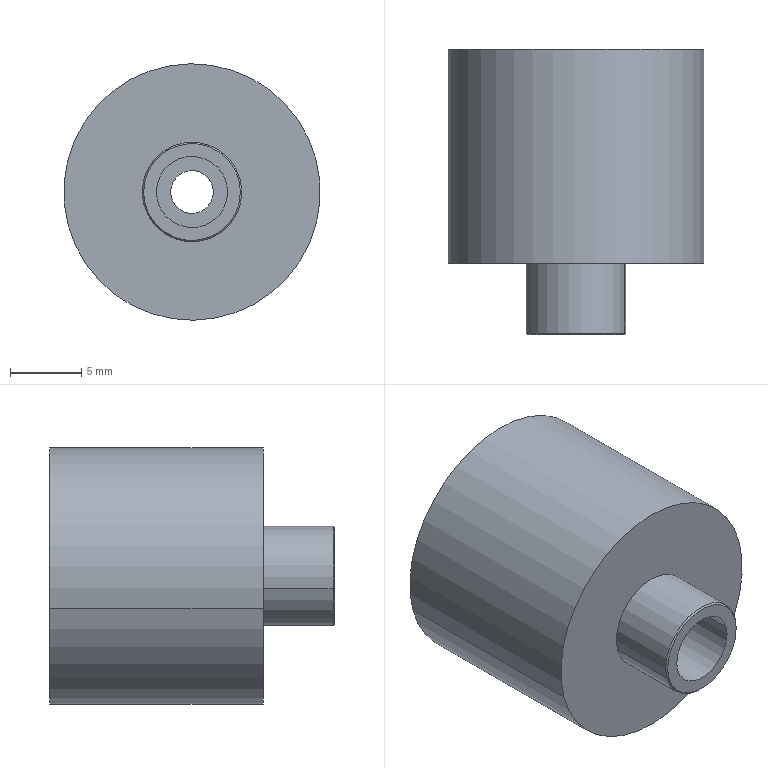Component | SolidWorks | WireFeedingConnector-1 | 1 solid | 19 faces | box 18 x 20 x 18 mm | volume 3059 mm3 | cylinder 10 | plane 5 | cone 4 | commonest cylinder face diameters 5 x2 10 x2 18 x2 7 x2 3 x2
build123d program:
from build123d import *

# Parameters (mm, degrees)
CHAMFER1_SIZE      = 0.1
CHAMFER2_SIZE      = 0.1
SKETCH1_R          = 2.5
CUT_EXTRUDE1_DEPTH = 7.5


with BuildPart() as part:
    # Sketch1_2 → Revolve1 (revolve)
    with BuildSketch(Plane.XY, mode=Mode.PRIVATE) as revolve1_sk:
        Polygon((-1.5, -5), (-3.5, -5), (-3.5, 0), (-9, 0), (-9, 15), (-5, 15), (-5, 5), (-1.5, 5), align=None)
    revolve(revolve1_sk.sketch.rotate(Axis((0, 18.5, 0), (0, -1, 0)), 270), axis=Axis((0, 18.5, 0), (0, -1, 0)))

    # Chamfer1
    chamfer1_edges = [part.edges().sort_by_distance(p)[0] for p in [
        (0, -5, -3.5),
    ]]
    chamfer(chamfer1_edges, length=CHAMFER1_SIZE)

    # Chamfer2
    chamfer2_edges = [part.edges().sort_by_distance(p)[0] for p in [
        (0, 15, -5),
    ]]
    chamfer(chamfer2_edges, length=CHAMFER2_SIZE)

    # Sketch1 → Cut-Extrude1 (cut)
    with BuildSketch(Plane.XZ.offset(5)):
        with Locations(Location((0, 0, 0), (0, 0, 270))):
            Circle(SKETCH1_R)
    extrude(amount=-CUT_EXTRUDE1_DEPTH, mode=Mode.SUBTRACT)


solid = part.part

# Placed as in the assembly
solid = solid.moved(Location((37.32, 90.506, 185), (0, 0, 0)))
STEP:
#1=COLOUR_RGB('',0.7922,0.8196,0.9333);
#2=FILL_AREA_STYLE_COLOUR('',#1);
#3=FILL_AREA_STYLE('',(#2));
#4=SURFACE_STYLE_FILL_AREA(#3);
#5=SURFACE_SIDE_STYLE('',(#4));
#6=SURFACE_STYLE_USAGE(.BOTH.,#5);
#7=PRESENTATION_STYLE_ASSIGNMENT((#6));
#8=CARTESIAN_POINT('',(1.564,3.662,7.309));
#9=VERTEX_POINT('',#8);
#10=CARTESIAN_POINT('',(1.374,3.662,7.258));
#11=VERTEX_POINT('',#10);
#12=CARTESIAN_POINT('',(1.469,3.662,7.283));
#13=DIRECTION('',(0.,-1.,0.));
#14=DIRECTION('',(-0.9666,0.,-0.2563));
#15=AXIS2_PLACEMENT_3D('',#12,#13,#14);
#16=CIRCLE('',#15,0.09843);
#17=EDGE_CURVE('',#9,#11,#16,.T.);
#18=ORIENTED_EDGE('',*,*,#17,.F.);
#19=CARTESIAN_POINT('',(1.564,3.366,7.309));
#20=VERTEX_POINT('',#19);
#21=CARTESIAN_POINT('',(1.564,3.662,7.309));
#22=DIRECTION('',(0.,-1.,0.));
#23=VECTOR('',#22,39.37);
#24=LINE('',#21,#23);
#25=EDGE_CURVE('',#9,#20,#24,.T.);
#26=ORIENTED_EDGE('',*,*,#25,.T.);
#27=CARTESIAN_POINT('',(1.374,3.366,7.258));
#28=VERTEX_POINT('',#27);
#29=CARTESIAN_POINT('',(1.469,3.366,7.283));
#30=DIRECTION('',(0.,-1.,0.));
#31=DIRECTION('',(-0.9666,0.,-0.2563));
#32=AXIS2_PLACEMENT_3D('',#29,#30,#31);
#33=CIRCLE('',#32,0.09843);
#34=EDGE_CURVE('',#20,#28,#33,.T.);
#35=ORIENTED_EDGE('',*,*,#34,.T.);
#36=CARTESIAN_POINT('',(1.374,3.662,7.258));
#37=DIRECTION('',(0.,-1.,0.));
#38=VECTOR('',#37,39.37);
#39=LINE('',#36,#38);
#40=EDGE_CURVE('',#11,#28,#39,.T.);
#41=ORIENTED_EDGE('',*,*,#40,.F.);
#42=EDGE_LOOP('',(#18,#26,#35,#41));
#43=FACE_OUTER_BOUND('',#42,.T.);
#44=CARTESIAN_POINT('',(1.469,3.662,7.283));
#45=DIRECTION('',(0.,-1.,0.));
#46=DIRECTION('',(-0.9666,0.,-0.2563));
#47=AXIS2_PLACEMENT_3D('',#44,#45,#46);
#48=CYLINDRICAL_SURFACE('',#47,0.09843);
#49=ADVANCED_FACE('',(#43),#48,.F.);
#50=CARTESIAN_POINT('',(1.279,4.15,7.233));
#51=VERTEX_POINT('',#50);
#52=CARTESIAN_POINT('',(1.66,4.15,7.334));
#53=VERTEX_POINT('',#52);
#54=CARTESIAN_POINT('',(1.469,4.15,7.283));
#55=DIRECTION('',(0.,1.,0.));
#56=DIRECTION('',(0.9666,0.,0.2563));
#57=AXIS2_PLACEMENT_3D('',#54,#55,#56);
#58=CIRCLE('',#57,0.1969);
#59=EDGE_CURVE('',#51,#53,#58,.T.);
#60=ORIENTED_EDGE('',*,*,#59,.F.);
#61=CARTESIAN_POINT('',(1.275,4.154,7.232));
#62=VERTEX_POINT('',#61);
#63=CARTESIAN_POINT('',(1.279,4.15,7.233));
#64=DIRECTION('',(-0.6835,0.7071,-0.1812));
#65=VECTOR('',#64,39.37);
#66=LINE('',#63,#65);
#67=EDGE_CURVE('',#51,#62,#66,.T.);
#68=ORIENTED_EDGE('',*,*,#67,.T.);
#69=CARTESIAN_POINT('',(1.663,4.154,7.335));
#70=VERTEX_POINT('',#69);
#71=CARTESIAN_POINT('',(1.469,4.154,7.283));
#72=DIRECTION('',(0.,-1.,0.));
#73=DIRECTION('',(0.9666,0.,0.2563));
#74=AXIS2_PLACEMENT_3D('',#71,#72,#73);
#75=CIRCLE('',#74,0.2008);
#76=EDGE_CURVE('',#70,#62,#75,.T.);
#77=ORIENTED_EDGE('',*,*,#76,.F.);
#78=CARTESIAN_POINT('',(1.66,4.15,7.334));
#79=DIRECTION('',(0.6835,0.7071,0.1812));
#80=VECTOR('',#79,39.37);
#81=LINE('',#78,#80);
#82=EDGE_CURVE('',#53,#70,#81,.T.);
#83=ORIENTED_EDGE('',*,*,#82,.F.);
#84=EDGE_LOOP('',(#60,#68,#77,#83));
#85=FACE_OUTER_BOUND('',#84,.T.);
#86=CARTESIAN_POINT('',(1.469,4.15,7.283));
#87=DIRECTION('',(0.,1.,0.));
#88=DIRECTION('',(0.9666,0.,0.2563));
#89=AXIS2_PLACEMENT_3D('',#86,#87,#88);
#90=CONICAL_SURFACE('',#89,0.1969,0.7854);
#91=ADVANCED_FACE('',(#85),#90,.F.);
#92=CARTESIAN_POINT('',(1.34,3.366,7.249));
#93=VERTEX_POINT('',#92);
#94=CARTESIAN_POINT('',(1.599,3.366,7.318));
#95=VERTEX_POINT('',#94);
#96=CARTESIAN_POINT('',(1.469,3.366,7.283));
#97=DIRECTION('',(0.,-1.,0.));
#98=DIRECTION('',(-0.9666,0.,-0.2563));
#99=AXIS2_PLACEMENT_3D('',#96,#97,#98);
#100=CIRCLE('',#99,0.1339);
#101=EDGE_CURVE('',#93,#95,#100,.T.);
#102=ORIENTED_EDGE('',*,*,#101,.F.);
#103=CARTESIAN_POINT('',(1.336,3.37,7.248));
#104=VERTEX_POINT('',#103);
#105=CARTESIAN_POINT('',(1.336,3.37,7.248));
#106=DIRECTION('',(-0.6835,0.7071,-0.1812));
#107=VECTOR('',#106,39.37);
#108=LINE('',#105,#107);
#109=EDGE_CURVE('',#93,#104,#108,.T.);
#110=ORIENTED_EDGE('',*,*,#109,.T.);
#111=CARTESIAN_POINT('',(1.602,3.37,7.319));
#112=VERTEX_POINT('',#111);
#113=CARTESIAN_POINT('',(1.469,3.37,7.283));
#114=DIRECTION('',(0.,1.,0.));
#115=DIRECTION('',(-0.9666,0.,-0.2563));
#116=AXIS2_PLACEMENT_3D('',#113,#114,#115);
#117=CIRCLE('',#116,0.1378);
#118=EDGE_CURVE('',#112,#104,#117,.T.);
#119=ORIENTED_EDGE('',*,*,#118,.F.);
#120=CARTESIAN_POINT('',(1.602,3.37,7.319));
#121=DIRECTION('',(0.6835,0.7071,0.1812));
#122=VECTOR('',#121,39.37);
#123=LINE('',#120,#122);
#124=EDGE_CURVE('',#95,#112,#123,.T.);
#125=ORIENTED_EDGE('',*,*,#124,.F.);
#126=EDGE_LOOP('',(#102,#110,#119,#125));
#127=FACE_OUTER_BOUND('',#126,.T.);
#128=CARTESIAN_POINT('',(1.469,3.37,7.283));
#129=DIRECTION('',(0.,1.,0.));
#130=DIRECTION('',(0.9666,0.,0.2563));
#131=AXIS2_PLACEMENT_3D('',#128,#129,#130);
#132=CONICAL_SURFACE('',#131,0.1378,0.7854);
#133=ADVANCED_FACE('',(#127),#132,.T.);
#134=CARTESIAN_POINT('',(1.279,3.76,7.233));
#135=VERTEX_POINT('',#134);
#136=CARTESIAN_POINT('',(1.66,3.76,7.334));
#137=VERTEX_POINT('',#136);
#138=CARTESIAN_POINT('',(1.469,3.76,7.283));
#139=DIRECTION('',(0.,1.,0.));
#140=DIRECTION('',(0.9666,0.,0.2563));
#141=AXIS2_PLACEMENT_3D('',#138,#139,#140);
#142=CIRCLE('',#141,0.1969);
#143=EDGE_CURVE('',#135,#137,#142,.T.);
#144=ORIENTED_EDGE('',*,*,#143,.F.);
#145=CARTESIAN_POINT('',(1.279,4.292,7.233));
#146=DIRECTION('',(0.,1.,0.));
#147=VECTOR('',#146,39.37);
#148=LINE('',#145,#147);
#149=EDGE_CURVE('',#135,#51,#148,.T.);
#150=ORIENTED_EDGE('',*,*,#149,.T.);
#151=ORIENTED_EDGE('',*,*,#59,.T.);
#152=CARTESIAN_POINT('',(1.66,4.292,7.334));
#153=DIRECTION('',(0.,1.,0.));
#154=VECTOR('',#153,39.37);
#155=LINE('',#152,#154);
#156=EDGE_CURVE('',#137,#53,#155,.T.);
#157=ORIENTED_EDGE('',*,*,#156,.F.);
#158=EDGE_LOOP('',(#144,#150,#151,#157));
#159=FACE_OUTER_BOUND('',#158,.T.);
#160=CARTESIAN_POINT('',(1.469,4.292,7.283));
#161=DIRECTION('',(0.,1.,0.));
#162=DIRECTION('',(0.9666,0.,0.2563));
#163=AXIS2_PLACEMENT_3D('',#160,#161,#162);
#164=CYLINDRICAL_SURFACE('',#163,0.1969);
#165=ADVANCED_FACE('',(#159),#164,.F.);
#166=CARTESIAN_POINT('',(1.812,3.563,7.374));
#167=VERTEX_POINT('',#166);
#168=CARTESIAN_POINT('',(1.127,3.563,7.193));
#169=VERTEX_POINT('',#168);
#170=CARTESIAN_POINT('',(1.469,3.563,7.283));
#171=DIRECTION('',(0.,1.,0.));
#172=DIRECTION('',(0.9666,0.,0.2563));
#173=AXIS2_PLACEMENT_3D('',#170,#171,#172);
#174=CIRCLE('',#173,0.3543);
#175=EDGE_CURVE('',#167,#169,#174,.T.);
#176=ORIENTED_EDGE('',*,*,#175,.T.);
#177=CARTESIAN_POINT('',(1.127,4.154,7.193));
#178=VERTEX_POINT('',#177);
#179=CARTESIAN_POINT('',(1.127,4.292,7.193));
#180=DIRECTION('',(0.,1.,0.));
#181=VECTOR('',#180,39.37);
#182=LINE('',#179,#181);
#183=EDGE_CURVE('',#169,#178,#182,.T.);
#184=ORIENTED_EDGE('',*,*,#183,.T.);
#185=CARTESIAN_POINT('',(1.812,4.154,7.374));
#186=VERTEX_POINT('',#185);
#187=CARTESIAN_POINT('',(1.469,4.154,7.283));
#188=DIRECTION('',(0.,1.,0.));
#189=DIRECTION('',(0.9666,0.,0.2563));
#190=AXIS2_PLACEMENT_3D('',#187,#188,#189);
#191=CIRCLE('',#190,0.3543);
#192=EDGE_CURVE('',#186,#178,#191,.T.);
#193=ORIENTED_EDGE('',*,*,#192,.F.);
#194=CARTESIAN_POINT('',(1.812,4.292,7.374));
#195=DIRECTION('',(0.,1.,0.));
#196=VECTOR('',#195,39.37);
#197=LINE('',#194,#196);
#198=EDGE_CURVE('',#167,#186,#197,.T.);
#199=ORIENTED_EDGE('',*,*,#198,.F.);
#200=EDGE_LOOP('',(#176,#184,#193,#199));
#201=FACE_OUTER_BOUND('',#200,.T.);
#202=CARTESIAN_POINT('',(1.469,4.292,7.283));
#203=DIRECTION('',(0.,1.,0.));
#204=DIRECTION('',(0.9666,0.,0.2563));
#205=AXIS2_PLACEMENT_3D('',#202,#203,#204);
#206=CYLINDRICAL_SURFACE('',#205,0.3543);
#207=ADVANCED_FACE('',(#201),#206,.T.);
#208=ORIENTED_EDGE('',*,*,#118,.T.);
#209=CARTESIAN_POINT('',(1.336,3.563,7.248));
#210=VERTEX_POINT('',#209);
#211=CARTESIAN_POINT('',(1.336,4.292,7.248));
#212=DIRECTION('',(0.,1.,0.));
#213=VECTOR('',#212,39.37);
#214=LINE('',#211,#213);
#215=EDGE_CURVE('',#104,#210,#214,.T.);
#216=ORIENTED_EDGE('',*,*,#215,.T.);
#217=CARTESIAN_POINT('',(1.602,3.563,7.319));
#218=VERTEX_POINT('',#217);
#219=CARTESIAN_POINT('',(1.469,3.563,7.283));
#220=DIRECTION('',(0.,1.,0.));
#221=DIRECTION('',(0.9666,0.,0.2563));
#222=AXIS2_PLACEMENT_3D('',#219,#220,#221);
#223=CIRCLE('',#222,0.1378);
#224=EDGE_CURVE('',#218,#210,#223,.T.);
#225=ORIENTED_EDGE('',*,*,#224,.F.);
#226=CARTESIAN_POINT('',(1.602,4.292,7.319));
#227=DIRECTION('',(0.,1.,0.));
#228=VECTOR('',#227,39.37);
#229=LINE('',#226,#228);
#230=EDGE_CURVE('',#112,#218,#229,.T.);
#231=ORIENTED_EDGE('',*,*,#230,.F.);
#232=EDGE_LOOP('',(#208,#216,#225,#231));
#233=FACE_OUTER_BOUND('',#232,.T.);
#234=CARTESIAN_POINT('',(1.469,4.292,7.283));
#235=DIRECTION('',(0.,1.,0.));
#236=DIRECTION('',(0.9666,0.,0.2563));
#237=AXIS2_PLACEMENT_3D('',#234,#235,#236);
#238=CYLINDRICAL_SURFACE('',#237,0.1378);
#239=ADVANCED_FACE('',(#233),#238,.T.);
#240=CARTESIAN_POINT('',(1.526,3.662,7.299));
#241=VERTEX_POINT('',#240);
#242=CARTESIAN_POINT('',(1.412,3.662,7.268));
#243=VERTEX_POINT('',#242);
#244=CARTESIAN_POINT('',(1.469,3.662,7.283));
#245=DIRECTION('',(0.,-1.,0.));
#246=DIRECTION('',(-0.9666,0.,-0.2563));
#247=AXIS2_PLACEMENT_3D('',#244,#245,#246);
#248=CIRCLE('',#247,0.05906);
#249=EDGE_CURVE('',#241,#243,#248,.T.);
#250=ORIENTED_EDGE('',*,*,#249,.T.);
#251=CARTESIAN_POINT('',(1.412,3.76,7.268));
#252=VERTEX_POINT('',#251);
#253=CARTESIAN_POINT('',(1.412,4.292,7.268));
#254=DIRECTION('',(0.,1.,0.));
#255=VECTOR('',#254,39.37);
#256=LINE('',#253,#255);
#257=EDGE_CURVE('',#243,#252,#256,.T.);
#258=ORIENTED_EDGE('',*,*,#257,.T.);
#259=CARTESIAN_POINT('',(1.526,3.76,7.299));
#260=VERTEX_POINT('',#259);
#261=CARTESIAN_POINT('',(1.469,3.76,7.283));
#262=DIRECTION('',(0.,1.,0.));
#263=DIRECTION('',(0.9666,0.,0.2563));
#264=AXIS2_PLACEMENT_3D('',#261,#262,#263);
#265=CIRCLE('',#264,0.05906);
#266=EDGE_CURVE('',#252,#260,#265,.T.);
#267=ORIENTED_EDGE('',*,*,#266,.T.);
#268=CARTESIAN_POINT('',(1.526,4.292,7.299));
#269=DIRECTION('',(0.,1.,0.));
#270=VECTOR('',#269,39.37);
#271=LINE('',#268,#270);
#272=EDGE_CURVE('',#241,#260,#271,.T.);
#273=ORIENTED_EDGE('',*,*,#272,.F.);
#274=EDGE_LOOP('',(#250,#258,#267,#273));
#275=FACE_OUTER_BOUND('',#274,.T.);
#276=CARTESIAN_POINT('',(1.469,4.292,7.283));
#277=DIRECTION('',(0.,1.,0.));
#278=DIRECTION('',(0.9666,0.,0.2563));
#279=AXIS2_PLACEMENT_3D('',#276,#277,#278);
#280=CYLINDRICAL_SURFACE('',#279,0.05906);
#281=ADVANCED_FACE('',(#275),#280,.F.);
#282=ORIENTED_EDGE('',*,*,#257,.F.);
#283=CARTESIAN_POINT('',(1.469,3.662,7.283));
#284=DIRECTION('',(0.,-1.,0.));
#285=DIRECTION('',(-0.9666,0.,-0.2563));
#286=AXIS2_PLACEMENT_3D('',#283,#284,#285);
#287=CIRCLE('',#286,0.05906);
#288=EDGE_CURVE('',#243,#241,#287,.T.);
#289=ORIENTED_EDGE('',*,*,#288,.T.);
#290=ORIENTED_EDGE('',*,*,#272,.T.);
#291=CARTESIAN_POINT('',(1.469,3.76,7.283));
#292=DIRECTION('',(0.,1.,0.));
#293=DIRECTION('',(0.9666,0.,0.2563));
#294=AXIS2_PLACEMENT_3D('',#291,#292,#293);
#295=CIRCLE('',#294,0.05906);
#296=EDGE_CURVE('',#260,#252,#295,.T.);
#297=ORIENTED_EDGE('',*,*,#296,.T.);
#298=EDGE_LOOP('',(#282,#289,#290,#297));
#299=FACE_OUTER_BOUND('',#298,.T.);
#300=CARTESIAN_POINT('',(1.469,4.292,7.283));
#301=DIRECTION('',(0.,1.,0.));
#302=DIRECTION('',(0.9666,0.,0.2563));
#303=AXIS2_PLACEMENT_3D('',#300,#301,#302);
#304=CYLINDRICAL_SURFACE('',#303,0.05906);
#305=ADVANCED_FACE('',(#299),#304,.F.);
#306=CARTESIAN_POINT('',(1.469,3.366,7.283));
#307=DIRECTION('',(0.,-1.,0.));
#308=DIRECTION('',(-0.9666,0.,-0.2563));
#309=AXIS2_PLACEMENT_3D('',#306,#307,#308);
#310=CIRCLE('',#309,0.09843);
#311=EDGE_CURVE('',#28,#20,#310,.T.);
#312=ORIENTED_EDGE('',*,*,#311,.F.);
#313=ORIENTED_EDGE('',*,*,#34,.F.);
#314=EDGE_LOOP('',(#312,#313));
#315=FACE_BOUND('',#314,.T.);
#316=CARTESIAN_POINT('',(1.469,3.366,7.283));
#317=DIRECTION('',(0.,-1.,0.));
#318=DIRECTION('',(-0.9666,0.,-0.2563));
#319=AXIS2_PLACEMENT_3D('',#316,#317,#318);
#320=CIRCLE('',#319,0.1339);
#321=EDGE_CURVE('',#95,#93,#320,.T.);
#322=ORIENTED_EDGE('',*,*,#321,.T.);
#323=ORIENTED_EDGE('',*,*,#101,.T.);
#324=EDGE_LOOP('',(#322,#323));
#325=FACE_OUTER_BOUND('',#324,.T.);
#326=CARTESIAN_POINT('',(1.454,3.366,7.341));
#327=DIRECTION('',(0.,-1.,0.));
#328=DIRECTION('',(-0.9666,0.,-0.2563));
#329=AXIS2_PLACEMENT_3D('',#326,#327,#328);
#330=PLANE('',#329);
#331=ADVANCED_FACE('',(#315,#325),#330,.T.);
#332=ORIENTED_EDGE('',*,*,#215,.F.);
#333=CARTESIAN_POINT('',(1.469,3.37,7.283));
#334=DIRECTION('',(0.,1.,0.));
#335=DIRECTION('',(-0.9666,0.,-0.2563));
#336=AXIS2_PLACEMENT_3D('',#333,#334,#335);
#337=CIRCLE('',#336,0.1378);
#338=EDGE_CURVE('',#104,#112,#337,.T.);
#339=ORIENTED_EDGE('',*,*,#338,.T.);
#340=ORIENTED_EDGE('',*,*,#230,.T.);
#341=CARTESIAN_POINT('',(1.469,3.563,7.283));
#342=DIRECTION('',(0.,1.,0.));
#343=DIRECTION('',(0.9666,0.,0.2563));
#344=AXIS2_PLACEMENT_3D('',#341,#342,#343);
#345=CIRCLE('',#344,0.1378);
#346=EDGE_CURVE('',#210,#218,#345,.T.);
#347=ORIENTED_EDGE('',*,*,#346,.F.);
#348=EDGE_LOOP('',(#332,#339,#340,#347));
#349=FACE_OUTER_BOUND('',#348,.T.);
#350=CARTESIAN_POINT('',(1.469,4.292,7.283));
#351=DIRECTION('',(0.,1.,0.));
#352=DIRECTION('',(0.9666,0.,0.2563));
#353=AXIS2_PLACEMENT_3D('',#350,#351,#352);
#354=CYLINDRICAL_SURFACE('',#353,0.1378);
#355=ADVANCED_FACE('',(#349),#354,.T.);
#356=ORIENTED_EDGE('',*,*,#224,.T.);
#357=ORIENTED_EDGE('',*,*,#346,.T.);
#358=EDGE_LOOP('',(#356,#357));
#359=FACE_BOUND('',#358,.T.);
#360=ORIENTED_EDGE('',*,*,#175,.F.);
#361=CARTESIAN_POINT('',(1.469,3.563,7.283));
#362=DIRECTION('',(0.,1.,0.));
#363=DIRECTION('',(0.9666,0.,0.2563));
#364=AXIS2_PLACEMENT_3D('',#361,#362,#363);
#365=CIRCLE('',#364,0.3543);
#366=EDGE_CURVE('',#169,#167,#365,.T.);
#367=ORIENTED_EDGE('',*,*,#366,.F.);
#368=EDGE_LOOP('',(#360,#367));
#369=FACE_OUTER_BOUND('',#368,.T.);
#370=CARTESIAN_POINT('',(1.434,3.563,7.417));
#371=DIRECTION('',(0.,-1.,0.));
#372=DIRECTION('',(-0.9666,0.,-0.2563));
#373=AXIS2_PLACEMENT_3D('',#370,#371,#372);
#374=PLANE('',#373);
#375=ADVANCED_FACE('',(#359,#369),#374,.T.);
#376=ORIENTED_EDGE('',*,*,#183,.F.);
#377=ORIENTED_EDGE('',*,*,#366,.T.);
#378=ORIENTED_EDGE('',*,*,#198,.T.);
#379=CARTESIAN_POINT('',(1.469,4.154,7.283));
#380=DIRECTION('',(0.,1.,0.));
#381=DIRECTION('',(0.9666,0.,0.2563));
#382=AXIS2_PLACEMENT_3D('',#379,#380,#381);
#383=CIRCLE('',#382,0.3543);
#384=EDGE_CURVE('',#178,#186,#383,.T.);
#385=ORIENTED_EDGE('',*,*,#384,.F.);
#386=EDGE_LOOP('',(#376,#377,#378,#385));
#387=FACE_OUTER_BOUND('',#386,.T.);
#388=CARTESIAN_POINT('',(1.469,4.292,7.283));
#389=DIRECTION('',(0.,1.,0.));
#390=DIRECTION('',(0.9666,0.,0.2563));
#391=AXIS2_PLACEMENT_3D('',#388,#389,#390);
#392=CYLINDRICAL_SURFACE('',#391,0.3543);
#393=ADVANCED_FACE('',(#387),#392,.T.);
#394=ORIENTED_EDGE('',*,*,#76,.T.);
#395=CARTESIAN_POINT('',(1.469,4.154,7.283));
#396=DIRECTION('',(0.,-1.,0.));
#397=DIRECTION('',(0.9666,0.,0.2563));
#398=AXIS2_PLACEMENT_3D('',#395,#396,#397);
#399=CIRCLE('',#398,0.2008);
#400=EDGE_CURVE('',#62,#70,#399,.T.);
#401=ORIENTED_EDGE('',*,*,#400,.T.);
#402=EDGE_LOOP('',(#394,#401));
#403=FACE_BOUND('',#402,.T.);
#404=ORIENTED_EDGE('',*,*,#192,.T.);
#405=ORIENTED_EDGE('',*,*,#384,.T.);
#406=EDGE_LOOP('',(#404,#405));
#407=FACE_OUTER_BOUND('',#406,.T.);
#408=CARTESIAN_POINT('',(1.378,4.154,7.626));
#409=DIRECTION('',(0.,1.,0.));
#410=DIRECTION('',(0.9666,0.,0.2563));
#411=AXIS2_PLACEMENT_3D('',#408,#409,#410);
#412=PLANE('',#411);
#413=ADVANCED_FACE('',(#403,#407),#412,.T.);
#414=ORIENTED_EDGE('',*,*,#149,.F.);
#415=CARTESIAN_POINT('',(1.469,3.76,7.283));
#416=DIRECTION('',(0.,1.,0.));
#417=DIRECTION('',(0.9666,0.,0.2563));
#418=AXIS2_PLACEMENT_3D('',#415,#416,#417);
#419=CIRCLE('',#418,0.1969);
#420=EDGE_CURVE('',#137,#135,#419,.T.);
#421=ORIENTED_EDGE('',*,*,#420,.F.);
#422=ORIENTED_EDGE('',*,*,#156,.T.);
#423=CARTESIAN_POINT('',(1.469,4.15,7.283));
#424=DIRECTION('',(0.,1.,0.));
#425=DIRECTION('',(0.9666,0.,0.2563));
#426=AXIS2_PLACEMENT_3D('',#423,#424,#425);
#427=CIRCLE('',#426,0.1969);
#428=EDGE_CURVE('',#53,#51,#427,.T.);
#429=ORIENTED_EDGE('',*,*,#428,.T.);
#430=EDGE_LOOP('',(#414,#421,#422,#429));
#431=FACE_OUTER_BOUND('',#430,.T.);
#432=CARTESIAN_POINT('',(1.469,4.292,7.283));
#433=DIRECTION('',(0.,1.,0.));
#434=DIRECTION('',(0.9666,0.,0.2563));
#435=AXIS2_PLACEMENT_3D('',#432,#433,#434);
#436=CYLINDRICAL_SURFACE('',#435,0.1969);
#437=ADVANCED_FACE('',(#431),#436,.F.);
#438=ORIENTED_EDGE('',*,*,#420,.T.);
#439=ORIENTED_EDGE('',*,*,#143,.T.);
#440=EDGE_LOOP('',(#438,#439));
#441=FACE_OUTER_BOUND('',#440,.T.);
#442=ORIENTED_EDGE('',*,*,#296,.F.);
#443=ORIENTED_EDGE('',*,*,#266,.F.);
#444=EDGE_LOOP('',(#442,#443));
#445=FACE_BOUND('',#444,.T.);
#446=CARTESIAN_POINT('',(1.419,3.76,7.474));
#447=DIRECTION('',(0.,1.,0.));
#448=DIRECTION('',(0.9666,0.,0.2563));
#449=AXIS2_PLACEMENT_3D('',#446,#447,#448);
#450=PLANE('',#449);
#451=ADVANCED_FACE('',(#441,#445),#450,.T.);
#452=ORIENTED_EDGE('',*,*,#109,.F.);
#453=ORIENTED_EDGE('',*,*,#321,.F.);
#454=ORIENTED_EDGE('',*,*,#124,.T.);
#455=ORIENTED_EDGE('',*,*,#338,.F.);
#456=EDGE_LOOP('',(#452,#453,#454,#455));
#457=FACE_OUTER_BOUND('',#456,.T.);
#458=CARTESIAN_POINT('',(1.469,3.37,7.283));
#459=DIRECTION('',(0.,1.,0.));
#460=DIRECTION('',(0.9666,0.,0.2563));
#461=AXIS2_PLACEMENT_3D('',#458,#459,#460);
#462=CONICAL_SURFACE('',#461,0.1378,0.7854);
#463=ADVANCED_FACE('',(#457),#462,.T.);
#464=ORIENTED_EDGE('',*,*,#67,.F.);
#465=ORIENTED_EDGE('',*,*,#428,.F.);
#466=ORIENTED_EDGE('',*,*,#82,.T.);
#467=ORIENTED_EDGE('',*,*,#400,.F.);
#468=EDGE_LOOP('',(#464,#465,#466,#467));
#469=FACE_OUTER_BOUND('',#468,.T.);
#470=CARTESIAN_POINT('',(1.469,4.15,7.283));
#471=DIRECTION('',(0.,1.,0.));
#472=DIRECTION('',(0.9666,0.,0.2563));
#473=AXIS2_PLACEMENT_3D('',#470,#471,#472);
#474=CONICAL_SURFACE('',#473,0.1969,0.7854);
#475=ADVANCED_FACE('',(#469),#474,.F.);
#476=ORIENTED_EDGE('',*,*,#25,.F.);
#477=CARTESIAN_POINT('',(1.469,3.662,7.283));
#478=DIRECTION('',(0.,-1.,0.));
#479=DIRECTION('',(-0.9666,0.,-0.2563));
#480=AXIS2_PLACEMENT_3D('',#477,#478,#479);
#481=CIRCLE('',#480,0.09843);
#482=EDGE_CURVE('',#11,#9,#481,.T.);
#483=ORIENTED_EDGE('',*,*,#482,.F.);
#484=ORIENTED_EDGE('',*,*,#40,.T.);
#485=ORIENTED_EDGE('',*,*,#311,.T.);
#486=EDGE_LOOP('',(#476,#483,#484,#485));
#487=FACE_OUTER_BOUND('',#486,.T.);
#488=CARTESIAN_POINT('',(1.469,3.662,7.283));
#489=DIRECTION('',(0.,-1.,0.));
#490=DIRECTION('',(-0.9666,0.,-0.2563));
#491=AXIS2_PLACEMENT_3D('',#488,#489,#490);
#492=CYLINDRICAL_SURFACE('',#491,0.09843);
#493=ADVANCED_FACE('',(#487),#492,.F.);
#494=ORIENTED_EDGE('',*,*,#249,.F.);
#495=ORIENTED_EDGE('',*,*,#288,.F.);
#496=EDGE_LOOP('',(#494,#495));
#497=FACE_BOUND('',#496,.T.);
#498=ORIENTED_EDGE('',*,*,#482,.T.);
#499=ORIENTED_EDGE('',*,*,#17,.T.);
#500=EDGE_LOOP('',(#498,#499));
#501=FACE_OUTER_BOUND('',#500,.T.);
#502=CARTESIAN_POINT('',(1.469,3.662,7.283));
#503=DIRECTION('',(0.,-1.,0.));
#504=DIRECTION('',(-0.9666,0.,-0.2563));
#505=AXIS2_PLACEMENT_3D('',#502,#503,#504);
#506=PLANE('',#505);
#507=ADVANCED_FACE('',(#497,#501),#506,.T.);
#508=CLOSED_SHELL('',(#49,#91,#133,#165,#207,#239,#281,#305,#331,#355,#375,#393,#413,#437,#451,#463,#475,#493,#507));
#509=MANIFOLD_SOLID_BREP('',#508);
#510=STYLED_ITEM('',(#7),#509);
#511=(LENGTH_UNIT()NAMED_UNIT(*)SI_UNIT($,.METRE.));
#512=LENGTH_MEASURE_WITH_UNIT(LENGTH_MEASURE(0.0254),#511);
#513=DIMENSIONAL_EXPONENTS(1.,0.,0.,0.,0.,0.,0.);
#514=(CONVERSION_BASED_UNIT('',#512)LENGTH_UNIT()NAMED_UNIT(#513));
#515=UNCERTAINTY_MEASURE_WITH_UNIT(LENGTH_MEASURE(0.00001),#514,'','');
#516=(NAMED_UNIT(*)PLANE_ANGLE_UNIT()SI_UNIT($,.RADIAN.));
#517=(NAMED_UNIT(*)SI_UNIT($,.STERADIAN.)SOLID_ANGLE_UNIT());
#518=(GEOMETRIC_REPRESENTATION_CONTEXT(3)GLOBAL_UNCERTAINTY_ASSIGNED_CONTEXT((#515))GLOBAL_UNIT_ASSIGNED_CONTEXT((#514,#516,#517))REPRESENTATION_CONTEXT('',''));
#519=MECHANICAL_DESIGN_GEOMETRIC_PRESENTATION_REPRESENTATION('',(#510),#518);
#520=CARTESIAN_POINT('',(0.,0.,0.));
#521=DIRECTION('',(0.,0.,1.));
#522=DIRECTION('',(1.,0.,0.));
#523=AXIS2_PLACEMENT_3D('',#520,#521,#522);
#524=(LENGTH_UNIT()NAMED_UNIT(*)SI_UNIT($,.METRE.));
#525=LENGTH_MEASURE_WITH_UNIT(LENGTH_MEASURE(0.0254),#524);
#526=DIMENSIONAL_EXPONENTS(1.,0.,0.,0.,0.,0.,0.);
#527=(CONVERSION_BASED_UNIT('',#525)LENGTH_UNIT()NAMED_UNIT(#526));
#528=UNCERTAINTY_MEASURE_WITH_UNIT(LENGTH_MEASURE(0.00001),#527,'','');
#529=(NAMED_UNIT(*)PLANE_ANGLE_UNIT()SI_UNIT($,.RADIAN.));
#530=(NAMED_UNIT(*)SI_UNIT($,.STERADIAN.)SOLID_ANGLE_UNIT());
#531=(GEOMETRIC_REPRESENTATION_CONTEXT(3)GLOBAL_UNCERTAINTY_ASSIGNED_CONTEXT((#528))GLOBAL_UNIT_ASSIGNED_CONTEXT((#527,#529,#530))REPRESENTATION_CONTEXT('',''));
#532=ADVANCED_BREP_SHAPE_REPRESENTATION('',(#509,#523),#531);
#533=PRESENTATION_LAYER_ASSIGNMENT('','',(#510));